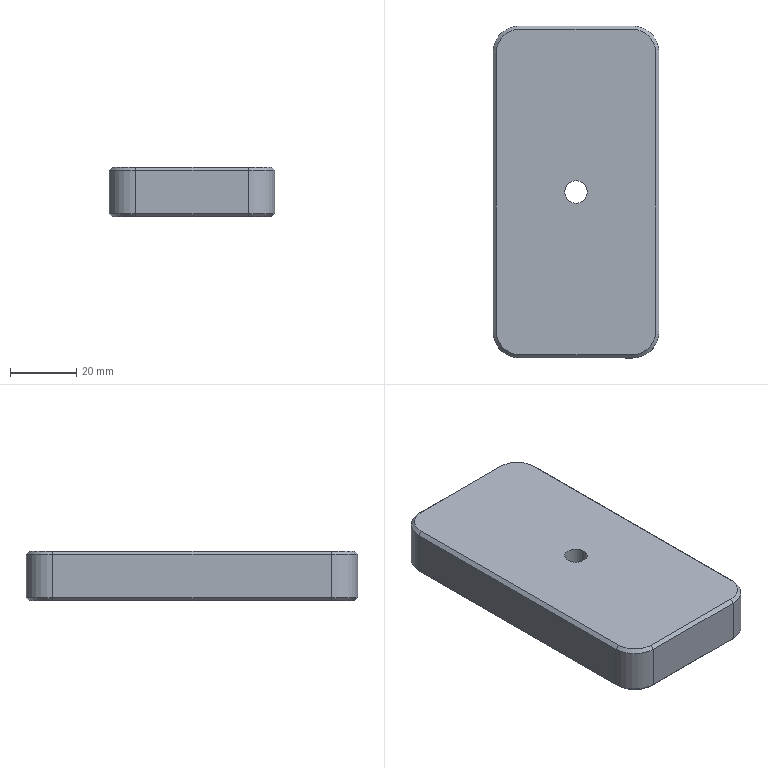Component | SolidWorks | 01-01FrameBody-1_02LowerRackSpacer-5 | 1 solid | 28 faces | box 50 x 100 x 15 mm | volume 73347 mm3 | plane 14 | cone 8 | cylinder 6 | commonest cylinder face diameters 16 x4 6.8 x2 | material 4040 Square Tube
build123d program:
from build123d import *

# Parameters (mm, degrees)
SKETCH1_W           = 50
SKETCH1_H           = 100
BOSS_EXTRUDE1_DEPTH = 15
M8_TAPPED_HOLE1_D   = 6.8
FILLET1_R           = 8
CHAMFER1_SIZE       = 1


with BuildPart() as part:
    # Sketch1 → Boss-Extrude1 (new body)
    with BuildSketch(Plane.XY):
        Rectangle(SKETCH1_W, SKETCH1_H)
    extrude(amount=BOSS_EXTRUDE1_DEPTH)

    # M8 Tapped Hole1 (through all)
    with Locations(Plane.XY.offset(15)):
        with Locations((0, 0)):
            Hole(M8_TAPPED_HOLE1_D / 2)

    # Fillet1
    fillet1_edges = [part.edges().sort_by_distance(p)[0] for p in [
        (25, -50, 7.5),
        (-25, -50, 7.5),
        (-25, 50, 7.5),
        (25, 50, 7.5),
    ]]
    fillet(fillet1_edges, radius=FILLET1_R)

    # Chamfer1
    chamfer1_edges = [part.edges().sort_by_distance(p)[0] for p in [
        (-25, 0, 0),
        (-25, 0, 15),
        (25, 0, 0),
        (0, -50, 0),
        (0, 50, 0),
        (22.657, -47.657, 0),
        (-22.657, -47.657, 0),
        (22.657, 47.657, 0),
        (-22.657, 47.657, 0),
        (0, 50, 15),
        (25, 0, 15),
        (0, -50, 15),
        (22.657, -47.657, 15),
        (-22.657, -47.657, 15),
        (22.657, 47.657, 15),
        (-22.657, 47.657, 15),
    ]]
    chamfer(chamfer1_edges, length=CHAMFER1_SIZE)


solid = part.part

# Placed as in the assembly
solid = solid.moved(Location((-25, 670, 625), (0, 0, 0)))
STEP:
#1=COLOUR_RGB('',0.7922,0.8196,0.9333);
#2=FILL_AREA_STYLE_COLOUR('',#1);
#3=FILL_AREA_STYLE('',(#2));
#4=SURFACE_STYLE_FILL_AREA(#3);
#5=SURFACE_SIDE_STYLE('',(#4));
#6=SURFACE_STYLE_USAGE(.BOTH.,#5);
#7=PRESENTATION_STYLE_ASSIGNMENT((#6));
#8=CARTESIAN_POINT('',(-1.118,26.378,25.197));
#9=VERTEX_POINT('',#8);
#10=CARTESIAN_POINT('',(-0.8504,26.378,25.197));
#11=VERTEX_POINT('',#10);
#12=CARTESIAN_POINT('',(-0.9843,26.378,25.197));
#13=DIRECTION('',(0.,-0.,-1.));
#14=DIRECTION('',(1.,0.,0.));
#15=AXIS2_PLACEMENT_3D('',#12,#13,#14);
#16=CIRCLE('',#15,0.1339);
#17=EDGE_CURVE('',#9,#11,#16,.T.);
#18=ORIENTED_EDGE('',*,*,#17,.F.);
#19=CARTESIAN_POINT('',(-1.118,26.378,24.606));
#20=VERTEX_POINT('',#19);
#21=CARTESIAN_POINT('',(-1.118,26.378,24.606));
#22=DIRECTION('',(0.,-0.,-1.));
#23=VECTOR('',#22,39.37);
#24=LINE('',#21,#23);
#25=EDGE_CURVE('',#9,#20,#24,.T.);
#26=ORIENTED_EDGE('',*,*,#25,.T.);
#27=CARTESIAN_POINT('',(-0.8504,26.378,24.606));
#28=VERTEX_POINT('',#27);
#29=CARTESIAN_POINT('',(-0.9843,26.378,24.606));
#30=DIRECTION('',(0.,-0.,-1.));
#31=DIRECTION('',(1.,0.,0.));
#32=AXIS2_PLACEMENT_3D('',#29,#30,#31);
#33=CIRCLE('',#32,0.1339);
#34=EDGE_CURVE('',#20,#28,#33,.T.);
#35=ORIENTED_EDGE('',*,*,#34,.T.);
#36=CARTESIAN_POINT('',(-0.8504,26.378,24.606));
#37=DIRECTION('',(0.,-0.,-1.));
#38=VECTOR('',#37,39.37);
#39=LINE('',#36,#38);
#40=EDGE_CURVE('',#11,#28,#39,.T.);
#41=ORIENTED_EDGE('',*,*,#40,.F.);
#42=EDGE_LOOP('',(#18,#26,#35,#41));
#43=FACE_OUTER_BOUND('',#42,.T.);
#44=CARTESIAN_POINT('',(-0.9843,26.378,24.606));
#45=DIRECTION('',(0.,-0.,-1.));
#46=DIRECTION('',(1.,0.,0.));
#47=AXIS2_PLACEMENT_3D('',#44,#45,#46);
#48=CYLINDRICAL_SURFACE('',#47,0.1339);
#49=ADVANCED_FACE('',(#43),#48,.F.);
#50=CARTESIAN_POINT('',(-0.,24.724,25.157));
#51=VERTEX_POINT('',#50);
#52=CARTESIAN_POINT('',(-0.,24.724,24.646));
#53=VERTEX_POINT('',#52);
#54=CARTESIAN_POINT('',(-0.,24.724,24.606));
#55=DIRECTION('',(0.,-0.,-1.));
#56=VECTOR('',#55,39.37);
#57=LINE('',#54,#56);
#58=EDGE_CURVE('',#51,#53,#57,.T.);
#59=ORIENTED_EDGE('',*,*,#58,.T.);
#60=CARTESIAN_POINT('',(-0.,28.031,24.646));
#61=VERTEX_POINT('',#60);
#62=CARTESIAN_POINT('',(-0.,28.031,24.646));
#63=DIRECTION('',(0.,1.,-0.));
#64=VECTOR('',#63,39.37);
#65=LINE('',#62,#64);
#66=EDGE_CURVE('',#53,#61,#65,.T.);
#67=ORIENTED_EDGE('',*,*,#66,.T.);
#68=CARTESIAN_POINT('',(-0.,28.031,25.157));
#69=VERTEX_POINT('',#68);
#70=CARTESIAN_POINT('',(-0.,28.031,24.606));
#71=DIRECTION('',(-0.,0.,1.));
#72=VECTOR('',#71,39.37);
#73=LINE('',#70,#72);
#74=EDGE_CURVE('',#61,#69,#73,.T.);
#75=ORIENTED_EDGE('',*,*,#74,.T.);
#76=CARTESIAN_POINT('',(-0.,24.409,25.157));
#77=DIRECTION('',(-0.,-1.,0.));
#78=VECTOR('',#77,39.37);
#79=LINE('',#76,#78);
#80=EDGE_CURVE('',#69,#51,#79,.T.);
#81=ORIENTED_EDGE('',*,*,#80,.T.);
#82=EDGE_LOOP('',(#59,#67,#75,#81));
#83=FACE_OUTER_BOUND('',#82,.T.);
#84=CARTESIAN_POINT('',(-0.,24.409,24.606));
#85=DIRECTION('',(-1.,0.,-0.));
#86=DIRECTION('',(0.,1.,-0.));
#87=AXIS2_PLACEMENT_3D('',#84,#85,#86);
#88=PLANE('',#87);
#89=ADVANCED_FACE('',(#83),#88,.F.);
#90=CARTESIAN_POINT('',(-1.654,24.409,25.157));
#91=VERTEX_POINT('',#90);
#92=CARTESIAN_POINT('',(-1.654,24.409,24.646));
#93=VERTEX_POINT('',#92);
#94=CARTESIAN_POINT('',(-1.654,24.409,24.606));
#95=DIRECTION('',(0.,-0.,-1.));
#96=VECTOR('',#95,39.37);
#97=LINE('',#94,#96);
#98=EDGE_CURVE('',#91,#93,#97,.T.);
#99=ORIENTED_EDGE('',*,*,#98,.T.);
#100=CARTESIAN_POINT('',(-0.315,24.409,24.646));
#101=VERTEX_POINT('',#100);
#102=CARTESIAN_POINT('',(-0.315,24.409,24.646));
#103=DIRECTION('',(1.,-0.,0.));
#104=VECTOR('',#103,39.37);
#105=LINE('',#102,#104);
#106=EDGE_CURVE('',#93,#101,#105,.T.);
#107=ORIENTED_EDGE('',*,*,#106,.T.);
#108=CARTESIAN_POINT('',(-0.315,24.409,25.157));
#109=VERTEX_POINT('',#108);
#110=CARTESIAN_POINT('',(-0.315,24.409,24.606));
#111=DIRECTION('',(-0.,0.,1.));
#112=VECTOR('',#111,39.37);
#113=LINE('',#110,#112);
#114=EDGE_CURVE('',#101,#109,#113,.T.);
#115=ORIENTED_EDGE('',*,*,#114,.T.);
#116=CARTESIAN_POINT('',(-1.969,24.409,25.157));
#117=DIRECTION('',(-1.,0.,-0.));
#118=VECTOR('',#117,39.37);
#119=LINE('',#116,#118);
#120=EDGE_CURVE('',#109,#91,#119,.T.);
#121=ORIENTED_EDGE('',*,*,#120,.T.);
#122=EDGE_LOOP('',(#99,#107,#115,#121));
#123=FACE_OUTER_BOUND('',#122,.T.);
#124=CARTESIAN_POINT('',(-1.969,24.409,24.606));
#125=DIRECTION('',(0.,1.,-0.));
#126=DIRECTION('',(-0.,0.,1.));
#127=AXIS2_PLACEMENT_3D('',#124,#125,#126);
#128=PLANE('',#127);
#129=ADVANCED_FACE('',(#123),#128,.F.);
#130=CARTESIAN_POINT('',(-1.969,28.031,25.157));
#131=VERTEX_POINT('',#130);
#132=CARTESIAN_POINT('',(-1.969,28.031,24.646));
#133=VERTEX_POINT('',#132);
#134=CARTESIAN_POINT('',(-1.969,28.031,24.606));
#135=DIRECTION('',(0.,-0.,-1.));
#136=VECTOR('',#135,39.37);
#137=LINE('',#134,#136);
#138=EDGE_CURVE('',#131,#133,#137,.T.);
#139=ORIENTED_EDGE('',*,*,#138,.T.);
#140=CARTESIAN_POINT('',(-1.969,24.724,24.646));
#141=VERTEX_POINT('',#140);
#142=CARTESIAN_POINT('',(-1.969,24.724,24.646));
#143=DIRECTION('',(-0.,-1.,0.));
#144=VECTOR('',#143,39.37);
#145=LINE('',#142,#144);
#146=EDGE_CURVE('',#133,#141,#145,.T.);
#147=ORIENTED_EDGE('',*,*,#146,.T.);
#148=CARTESIAN_POINT('',(-1.969,24.724,25.157));
#149=VERTEX_POINT('',#148);
#150=CARTESIAN_POINT('',(-1.969,24.724,24.606));
#151=DIRECTION('',(-0.,0.,1.));
#152=VECTOR('',#151,39.37);
#153=LINE('',#150,#152);
#154=EDGE_CURVE('',#141,#149,#153,.T.);
#155=ORIENTED_EDGE('',*,*,#154,.T.);
#156=CARTESIAN_POINT('',(-1.969,24.409,25.157));
#157=DIRECTION('',(0.,1.,-0.));
#158=VECTOR('',#157,39.37);
#159=LINE('',#156,#158);
#160=EDGE_CURVE('',#149,#131,#159,.T.);
#161=ORIENTED_EDGE('',*,*,#160,.T.);
#162=EDGE_LOOP('',(#139,#147,#155,#161));
#163=FACE_OUTER_BOUND('',#162,.T.);
#164=CARTESIAN_POINT('',(-1.969,24.409,24.606));
#165=DIRECTION('',(1.,-0.,0.));
#166=DIRECTION('',(-0.,-1.,0.));
#167=AXIS2_PLACEMENT_3D('',#164,#165,#166);
#168=PLANE('',#167);
#169=ADVANCED_FACE('',(#163),#168,.F.);
#170=CARTESIAN_POINT('',(-0.315,28.346,25.157));
#171=VERTEX_POINT('',#170);
#172=CARTESIAN_POINT('',(-0.315,28.346,24.646));
#173=VERTEX_POINT('',#172);
#174=CARTESIAN_POINT('',(-0.315,28.346,24.606));
#175=DIRECTION('',(0.,-0.,-1.));
#176=VECTOR('',#175,39.37);
#177=LINE('',#174,#176);
#178=EDGE_CURVE('',#171,#173,#177,.T.);
#179=ORIENTED_EDGE('',*,*,#178,.T.);
#180=CARTESIAN_POINT('',(-1.654,28.346,24.646));
#181=VERTEX_POINT('',#180);
#182=CARTESIAN_POINT('',(-1.654,28.346,24.646));
#183=DIRECTION('',(-1.,0.,-0.));
#184=VECTOR('',#183,39.37);
#185=LINE('',#182,#184);
#186=EDGE_CURVE('',#173,#181,#185,.T.);
#187=ORIENTED_EDGE('',*,*,#186,.T.);
#188=CARTESIAN_POINT('',(-1.654,28.346,25.157));
#189=VERTEX_POINT('',#188);
#190=CARTESIAN_POINT('',(-1.654,28.346,24.606));
#191=DIRECTION('',(-0.,0.,1.));
#192=VECTOR('',#191,39.37);
#193=LINE('',#190,#192);
#194=EDGE_CURVE('',#181,#189,#193,.T.);
#195=ORIENTED_EDGE('',*,*,#194,.T.);
#196=CARTESIAN_POINT('',(-1.969,28.346,25.157));
#197=DIRECTION('',(1.,-0.,0.));
#198=VECTOR('',#197,39.37);
#199=LINE('',#196,#198);
#200=EDGE_CURVE('',#189,#171,#199,.T.);
#201=ORIENTED_EDGE('',*,*,#200,.T.);
#202=EDGE_LOOP('',(#179,#187,#195,#201));
#203=FACE_OUTER_BOUND('',#202,.T.);
#204=CARTESIAN_POINT('',(-1.969,28.346,24.606));
#205=DIRECTION('',(-0.,-1.,0.));
#206=DIRECTION('',(0.,-0.,-1.));
#207=AXIS2_PLACEMENT_3D('',#204,#205,#206);
#208=PLANE('',#207);
#209=ADVANCED_FACE('',(#203),#208,.F.);
#210=CARTESIAN_POINT('',(-1.654,28.307,24.606));
#211=VERTEX_POINT('',#210);
#212=CARTESIAN_POINT('',(-0.315,28.307,24.606));
#213=VERTEX_POINT('',#212);
#214=CARTESIAN_POINT('',(-0.315,28.307,24.606));
#215=DIRECTION('',(1.,-0.,0.));
#216=VECTOR('',#215,39.37);
#217=LINE('',#214,#216);
#218=EDGE_CURVE('',#211,#213,#217,.T.);
#219=ORIENTED_EDGE('',*,*,#218,.T.);
#220=CARTESIAN_POINT('',(-0.03937,28.031,24.606));
#221=VERTEX_POINT('',#220);
#222=CARTESIAN_POINT('',(-0.315,28.031,24.606));
#223=DIRECTION('',(0.,-0.,-1.));
#224=DIRECTION('',(1.,0.,0.));
#225=AXIS2_PLACEMENT_3D('',#222,#223,#224);
#226=CIRCLE('',#225,0.2756);
#227=EDGE_CURVE('',#213,#221,#226,.T.);
#228=ORIENTED_EDGE('',*,*,#227,.T.);
#229=CARTESIAN_POINT('',(-0.03937,24.724,24.606));
#230=VERTEX_POINT('',#229);
#231=CARTESIAN_POINT('',(-0.03937,24.724,24.606));
#232=DIRECTION('',(-0.,-1.,0.));
#233=VECTOR('',#232,39.37);
#234=LINE('',#231,#233);
#235=EDGE_CURVE('',#221,#230,#234,.T.);
#236=ORIENTED_EDGE('',*,*,#235,.T.);
#237=CARTESIAN_POINT('',(-0.315,24.449,24.606));
#238=VERTEX_POINT('',#237);
#239=CARTESIAN_POINT('',(-0.315,24.724,24.606));
#240=DIRECTION('',(0.,-0.,-1.));
#241=DIRECTION('',(1.,0.,0.));
#242=AXIS2_PLACEMENT_3D('',#239,#240,#241);
#243=CIRCLE('',#242,0.2756);
#244=EDGE_CURVE('',#230,#238,#243,.T.);
#245=ORIENTED_EDGE('',*,*,#244,.T.);
#246=CARTESIAN_POINT('',(-1.654,24.449,24.606));
#247=VERTEX_POINT('',#246);
#248=CARTESIAN_POINT('',(-1.654,24.449,24.606));
#249=DIRECTION('',(-1.,0.,-0.));
#250=VECTOR('',#249,39.37);
#251=LINE('',#248,#250);
#252=EDGE_CURVE('',#238,#247,#251,.T.);
#253=ORIENTED_EDGE('',*,*,#252,.T.);
#254=CARTESIAN_POINT('',(-1.929,24.724,24.606));
#255=VERTEX_POINT('',#254);
#256=CARTESIAN_POINT('',(-1.654,24.724,24.606));
#257=DIRECTION('',(0.,-0.,-1.));
#258=DIRECTION('',(1.,0.,0.));
#259=AXIS2_PLACEMENT_3D('',#256,#257,#258);
#260=CIRCLE('',#259,0.2756);
#261=EDGE_CURVE('',#247,#255,#260,.T.);
#262=ORIENTED_EDGE('',*,*,#261,.T.);
#263=CARTESIAN_POINT('',(-1.929,28.031,24.606));
#264=VERTEX_POINT('',#263);
#265=CARTESIAN_POINT('',(-1.929,28.031,24.606));
#266=DIRECTION('',(0.,1.,-0.));
#267=VECTOR('',#266,39.37);
#268=LINE('',#265,#267);
#269=EDGE_CURVE('',#255,#264,#268,.T.);
#270=ORIENTED_EDGE('',*,*,#269,.T.);
#271=CARTESIAN_POINT('',(-1.654,28.031,24.606));
#272=DIRECTION('',(0.,-0.,-1.));
#273=DIRECTION('',(1.,0.,0.));
#274=AXIS2_PLACEMENT_3D('',#271,#272,#273);
#275=CIRCLE('',#274,0.2756);
#276=EDGE_CURVE('',#264,#211,#275,.T.);
#277=ORIENTED_EDGE('',*,*,#276,.T.);
#278=EDGE_LOOP('',(#219,#228,#236,#245,#253,#262,#270,#277));
#279=FACE_OUTER_BOUND('',#278,.T.);
#280=CARTESIAN_POINT('',(-0.9843,26.378,24.606));
#281=DIRECTION('',(0.,-0.,-1.));
#282=DIRECTION('',(1.,0.,0.));
#283=AXIS2_PLACEMENT_3D('',#280,#281,#282);
#284=CIRCLE('',#283,0.1339);
#285=EDGE_CURVE('',#28,#20,#284,.T.);
#286=ORIENTED_EDGE('',*,*,#285,.F.);
#287=ORIENTED_EDGE('',*,*,#34,.F.);
#288=EDGE_LOOP('',(#286,#287));
#289=FACE_BOUND('',#288,.T.);
#290=CARTESIAN_POINT('',(-0.,28.346,24.606));
#291=DIRECTION('',(0.,-0.,-1.));
#292=DIRECTION('',(1.,-0.,0.));
#293=AXIS2_PLACEMENT_3D('',#290,#291,#292);
#294=PLANE('',#293);
#295=ADVANCED_FACE('',(#279,#289),#294,.T.);
#296=CARTESIAN_POINT('',(-1.654,24.449,25.197));
#297=VERTEX_POINT('',#296);
#298=CARTESIAN_POINT('',(-0.315,24.449,25.197));
#299=VERTEX_POINT('',#298);
#300=CARTESIAN_POINT('',(-0.,24.449,25.197));
#301=DIRECTION('',(1.,-0.,0.));
#302=VECTOR('',#301,39.37);
#303=LINE('',#300,#302);
#304=EDGE_CURVE('',#297,#299,#303,.T.);
#305=ORIENTED_EDGE('',*,*,#304,.T.);
#306=CARTESIAN_POINT('',(-0.03937,24.724,25.197));
#307=VERTEX_POINT('',#306);
#308=CARTESIAN_POINT('',(-0.315,24.724,25.197));
#309=DIRECTION('',(-0.,0.,1.));
#310=DIRECTION('',(1.,0.,0.));
#311=AXIS2_PLACEMENT_3D('',#308,#309,#310);
#312=CIRCLE('',#311,0.2756);
#313=EDGE_CURVE('',#299,#307,#312,.T.);
#314=ORIENTED_EDGE('',*,*,#313,.T.);
#315=CARTESIAN_POINT('',(-0.03937,28.031,25.197));
#316=VERTEX_POINT('',#315);
#317=CARTESIAN_POINT('',(-0.03937,28.346,25.197));
#318=DIRECTION('',(0.,1.,-0.));
#319=VECTOR('',#318,39.37);
#320=LINE('',#317,#319);
#321=EDGE_CURVE('',#307,#316,#320,.T.);
#322=ORIENTED_EDGE('',*,*,#321,.T.);
#323=CARTESIAN_POINT('',(-0.315,28.307,25.197));
#324=VERTEX_POINT('',#323);
#325=CARTESIAN_POINT('',(-0.315,28.031,25.197));
#326=DIRECTION('',(-0.,0.,1.));
#327=DIRECTION('',(1.,0.,0.));
#328=AXIS2_PLACEMENT_3D('',#325,#326,#327);
#329=CIRCLE('',#328,0.2756);
#330=EDGE_CURVE('',#316,#324,#329,.T.);
#331=ORIENTED_EDGE('',*,*,#330,.T.);
#332=CARTESIAN_POINT('',(-1.654,28.307,25.197));
#333=VERTEX_POINT('',#332);
#334=CARTESIAN_POINT('',(-0.,28.307,25.197));
#335=DIRECTION('',(-1.,0.,-0.));
#336=VECTOR('',#335,39.37);
#337=LINE('',#334,#336);
#338=EDGE_CURVE('',#324,#333,#337,.T.);
#339=ORIENTED_EDGE('',*,*,#338,.T.);
#340=CARTESIAN_POINT('',(-1.929,28.031,25.197));
#341=VERTEX_POINT('',#340);
#342=CARTESIAN_POINT('',(-1.654,28.031,25.197));
#343=DIRECTION('',(-0.,0.,1.));
#344=DIRECTION('',(1.,0.,0.));
#345=AXIS2_PLACEMENT_3D('',#342,#343,#344);
#346=CIRCLE('',#345,0.2756);
#347=EDGE_CURVE('',#333,#341,#346,.T.);
#348=ORIENTED_EDGE('',*,*,#347,.T.);
#349=CARTESIAN_POINT('',(-1.929,24.724,25.197));
#350=VERTEX_POINT('',#349);
#351=CARTESIAN_POINT('',(-1.929,28.346,25.197));
#352=DIRECTION('',(-0.,-1.,0.));
#353=VECTOR('',#352,39.37);
#354=LINE('',#351,#353);
#355=EDGE_CURVE('',#341,#350,#354,.T.);
#356=ORIENTED_EDGE('',*,*,#355,.T.);
#357=CARTESIAN_POINT('',(-1.654,24.724,25.197));
#358=DIRECTION('',(-0.,0.,1.));
#359=DIRECTION('',(1.,0.,0.));
#360=AXIS2_PLACEMENT_3D('',#357,#358,#359);
#361=CIRCLE('',#360,0.2756);
#362=EDGE_CURVE('',#350,#297,#361,.T.);
#363=ORIENTED_EDGE('',*,*,#362,.T.);
#364=EDGE_LOOP('',(#305,#314,#322,#331,#339,#348,#356,#363));
#365=FACE_OUTER_BOUND('',#364,.T.);
#366=CARTESIAN_POINT('',(-0.9843,26.378,25.197));
#367=DIRECTION('',(0.,-0.,-1.));
#368=DIRECTION('',(1.,0.,0.));
#369=AXIS2_PLACEMENT_3D('',#366,#367,#368);
#370=CIRCLE('',#369,0.1339);
#371=EDGE_CURVE('',#11,#9,#370,.T.);
#372=ORIENTED_EDGE('',*,*,#371,.T.);
#373=ORIENTED_EDGE('',*,*,#17,.T.);
#374=EDGE_LOOP('',(#372,#373));
#375=FACE_BOUND('',#374,.T.);
#376=CARTESIAN_POINT('',(-0.,28.346,25.197));
#377=DIRECTION('',(0.,-0.,-1.));
#378=DIRECTION('',(1.,-0.,0.));
#379=AXIS2_PLACEMENT_3D('',#376,#377,#378);
#380=PLANE('',#379);
#381=ADVANCED_FACE('',(#365,#375),#380,.F.);
#382=ORIENTED_EDGE('',*,*,#25,.F.);
#383=ORIENTED_EDGE('',*,*,#371,.F.);
#384=ORIENTED_EDGE('',*,*,#40,.T.);
#385=ORIENTED_EDGE('',*,*,#285,.T.);
#386=EDGE_LOOP('',(#382,#383,#384,#385));
#387=FACE_OUTER_BOUND('',#386,.T.);
#388=CARTESIAN_POINT('',(-0.9843,26.378,24.606));
#389=DIRECTION('',(0.,-0.,-1.));
#390=DIRECTION('',(1.,0.,0.));
#391=AXIS2_PLACEMENT_3D('',#388,#389,#390);
#392=CYLINDRICAL_SURFACE('',#391,0.1339);
#393=ADVANCED_FACE('',(#387),#392,.F.);
#394=ORIENTED_EDGE('',*,*,#154,.F.);
#395=CARTESIAN_POINT('',(-1.654,24.724,24.646));
#396=DIRECTION('',(-0.,0.,1.));
#397=DIRECTION('',(1.,0.,0.));
#398=AXIS2_PLACEMENT_3D('',#395,#396,#397);
#399=CIRCLE('',#398,0.315);
#400=EDGE_CURVE('',#141,#93,#399,.T.);
#401=ORIENTED_EDGE('',*,*,#400,.T.);
#402=ORIENTED_EDGE('',*,*,#98,.F.);
#403=CARTESIAN_POINT('',(-1.654,24.724,25.157));
#404=DIRECTION('',(0.,-0.,-1.));
#405=DIRECTION('',(1.,0.,0.));
#406=AXIS2_PLACEMENT_3D('',#403,#404,#405);
#407=CIRCLE('',#406,0.315);
#408=EDGE_CURVE('',#91,#149,#407,.T.);
#409=ORIENTED_EDGE('',*,*,#408,.T.);
#410=EDGE_LOOP('',(#394,#401,#402,#409));
#411=FACE_OUTER_BOUND('',#410,.T.);
#412=CARTESIAN_POINT('',(-1.654,24.724,24.606));
#413=DIRECTION('',(-0.,0.,1.));
#414=DIRECTION('',(-1.,0.,0.));
#415=AXIS2_PLACEMENT_3D('',#412,#413,#414);
#416=CYLINDRICAL_SURFACE('',#415,0.315);
#417=ADVANCED_FACE('',(#411),#416,.T.);
#418=ORIENTED_EDGE('',*,*,#114,.F.);
#419=CARTESIAN_POINT('',(-0.315,24.724,24.646));
#420=DIRECTION('',(-0.,0.,1.));
#421=DIRECTION('',(1.,0.,0.));
#422=AXIS2_PLACEMENT_3D('',#419,#420,#421);
#423=CIRCLE('',#422,0.315);
#424=EDGE_CURVE('',#101,#53,#423,.T.);
#425=ORIENTED_EDGE('',*,*,#424,.T.);
#426=ORIENTED_EDGE('',*,*,#58,.F.);
#427=CARTESIAN_POINT('',(-0.315,24.724,25.157));
#428=DIRECTION('',(0.,-0.,-1.));
#429=DIRECTION('',(1.,0.,0.));
#430=AXIS2_PLACEMENT_3D('',#427,#428,#429);
#431=CIRCLE('',#430,0.315);
#432=EDGE_CURVE('',#51,#109,#431,.T.);
#433=ORIENTED_EDGE('',*,*,#432,.T.);
#434=EDGE_LOOP('',(#418,#425,#426,#433));
#435=FACE_OUTER_BOUND('',#434,.T.);
#436=CARTESIAN_POINT('',(-0.315,24.724,24.606));
#437=DIRECTION('',(-0.,0.,1.));
#438=DIRECTION('',(-1.,0.,0.));
#439=AXIS2_PLACEMENT_3D('',#436,#437,#438);
#440=CYLINDRICAL_SURFACE('',#439,0.315);
#441=ADVANCED_FACE('',(#435),#440,.T.);
#442=ORIENTED_EDGE('',*,*,#194,.F.);
#443=CARTESIAN_POINT('',(-1.654,28.031,24.646));
#444=DIRECTION('',(-0.,0.,1.));
#445=DIRECTION('',(1.,0.,0.));
#446=AXIS2_PLACEMENT_3D('',#443,#444,#445);
#447=CIRCLE('',#446,0.315);
#448=EDGE_CURVE('',#181,#133,#447,.T.);
#449=ORIENTED_EDGE('',*,*,#448,.T.);
#450=ORIENTED_EDGE('',*,*,#138,.F.);
#451=CARTESIAN_POINT('',(-1.654,28.031,25.157));
#452=DIRECTION('',(0.,-0.,-1.));
#453=DIRECTION('',(1.,0.,0.));
#454=AXIS2_PLACEMENT_3D('',#451,#452,#453);
#455=CIRCLE('',#454,0.315);
#456=EDGE_CURVE('',#131,#189,#455,.T.);
#457=ORIENTED_EDGE('',*,*,#456,.T.);
#458=EDGE_LOOP('',(#442,#449,#450,#457));
#459=FACE_OUTER_BOUND('',#458,.T.);
#460=CARTESIAN_POINT('',(-1.654,28.031,24.606));
#461=DIRECTION('',(-0.,0.,1.));
#462=DIRECTION('',(-1.,0.,0.));
#463=AXIS2_PLACEMENT_3D('',#460,#461,#462);
#464=CYLINDRICAL_SURFACE('',#463,0.315);
#465=ADVANCED_FACE('',(#459),#464,.T.);
#466=ORIENTED_EDGE('',*,*,#74,.F.);
#467=CARTESIAN_POINT('',(-0.315,28.031,24.646));
#468=DIRECTION('',(-0.,0.,1.));
#469=DIRECTION('',(1.,0.,0.));
#470=AXIS2_PLACEMENT_3D('',#467,#468,#469);
#471=CIRCLE('',#470,0.315);
#472=EDGE_CURVE('',#61,#173,#471,.T.);
#473=ORIENTED_EDGE('',*,*,#472,.T.);
#474=ORIENTED_EDGE('',*,*,#178,.F.);
#475=CARTESIAN_POINT('',(-0.315,28.031,25.157));
#476=DIRECTION('',(0.,-0.,-1.));
#477=DIRECTION('',(1.,0.,0.));
#478=AXIS2_PLACEMENT_3D('',#475,#476,#477);
#479=CIRCLE('',#478,0.315);
#480=EDGE_CURVE('',#171,#69,#479,.T.);
#481=ORIENTED_EDGE('',*,*,#480,.T.);
#482=EDGE_LOOP('',(#466,#473,#474,#481));
#483=FACE_OUTER_BOUND('',#482,.T.);
#484=CARTESIAN_POINT('',(-0.315,28.031,24.606));
#485=DIRECTION('',(-0.,0.,1.));
#486=DIRECTION('',(-1.,0.,0.));
#487=AXIS2_PLACEMENT_3D('',#484,#485,#486);
#488=CYLINDRICAL_SURFACE('',#487,0.315);
#489=ADVANCED_FACE('',(#483),#488,.T.);
#490=CARTESIAN_POINT('',(-1.654,24.409,24.646));
#491=DIRECTION('',(0.,0.7071,-0.7071));
#492=VECTOR('',#491,39.37);
#493=LINE('',#490,#492);
#494=EDGE_CURVE('',#93,#247,#493,.T.);
#495=ORIENTED_EDGE('',*,*,#494,.F.);
#496=ORIENTED_EDGE('',*,*,#400,.F.);
#497=CARTESIAN_POINT('',(-1.929,24.724,24.606));
#498=DIRECTION('',(-0.7071,0.,0.7071));
#499=VECTOR('',#498,39.37);
#500=LINE('',#497,#499);
#501=EDGE_CURVE('',#255,#141,#500,.T.);
#502=ORIENTED_EDGE('',*,*,#501,.F.);
#503=ORIENTED_EDGE('',*,*,#261,.F.);
#504=EDGE_LOOP('',(#495,#496,#502,#503));
#505=FACE_OUTER_BOUND('',#504,.T.);
#506=CARTESIAN_POINT('',(-1.654,24.724,24.606));
#507=DIRECTION('',(-0.,0.,1.));
#508=DIRECTION('',(-1.,0.,0.));
#509=AXIS2_PLACEMENT_3D('',#506,#507,#508);
#510=CONICAL_SURFACE('',#509,0.2756,0.7854);
#511=ADVANCED_FACE('',(#505),#510,.T.);
#512=ORIENTED_EDGE('',*,*,#501,.T.);
#513=ORIENTED_EDGE('',*,*,#146,.F.);
#514=CARTESIAN_POINT('',(-1.929,28.031,24.606));
#515=DIRECTION('',(-0.7071,0.,0.7071));
#516=VECTOR('',#515,39.37);
#517=LINE('',#514,#516);
#518=EDGE_CURVE('',#264,#133,#517,.T.);
#519=ORIENTED_EDGE('',*,*,#518,.F.);
#520=ORIENTED_EDGE('',*,*,#269,.F.);
#521=EDGE_LOOP('',(#512,#513,#519,#520));
#522=FACE_OUTER_BOUND('',#521,.T.);
#523=CARTESIAN_POINT('',(-1.929,28.346,24.606));
#524=DIRECTION('',(-0.7071,0.,-0.7071));
#525=DIRECTION('',(0.7071,-0.,-0.7071));
#526=AXIS2_PLACEMENT_3D('',#523,#524,#525);
#527=PLANE('',#526);
#528=ADVANCED_FACE('',(#522),#527,.T.);
#529=ORIENTED_EDGE('',*,*,#494,.T.);
#530=ORIENTED_EDGE('',*,*,#252,.F.);
#531=CARTESIAN_POINT('',(-0.315,24.409,24.646));
#532=DIRECTION('',(0.,0.7071,-0.7071));
#533=VECTOR('',#532,39.37);
#534=LINE('',#531,#533);
#535=EDGE_CURVE('',#101,#238,#534,.T.);
#536=ORIENTED_EDGE('',*,*,#535,.F.);
#537=ORIENTED_EDGE('',*,*,#106,.F.);
#538=EDGE_LOOP('',(#529,#530,#536,#537));
#539=FACE_OUTER_BOUND('',#538,.T.);
#540=CARTESIAN_POINT('',(-0.,24.449,24.606));
#541=DIRECTION('',(-0.,-0.7071,-0.7071));
#542=DIRECTION('',(0.,0.7071,-0.7071));
#543=AXIS2_PLACEMENT_3D('',#540,#541,#542);
#544=PLANE('',#543);
#545=ADVANCED_FACE('',(#539),#544,.T.);
#546=ORIENTED_EDGE('',*,*,#518,.T.);
#547=ORIENTED_EDGE('',*,*,#448,.F.);
#548=CARTESIAN_POINT('',(-1.654,28.307,24.606));
#549=DIRECTION('',(0.,0.7071,0.7071));
#550=VECTOR('',#549,39.37);
#551=LINE('',#548,#550);
#552=EDGE_CURVE('',#211,#181,#551,.T.);
#553=ORIENTED_EDGE('',*,*,#552,.F.);
#554=ORIENTED_EDGE('',*,*,#276,.F.);
#555=EDGE_LOOP('',(#546,#547,#553,#554));
#556=FACE_OUTER_BOUND('',#555,.T.);
#557=CARTESIAN_POINT('',(-1.654,28.031,24.606));
#558=DIRECTION('',(-0.,0.,1.));
#559=DIRECTION('',(-1.,0.,0.));
#560=AXIS2_PLACEMENT_3D('',#557,#558,#559);
#561=CONICAL_SURFACE('',#560,0.2756,0.7854);
#562=ADVANCED_FACE('',(#556),#561,.T.);
#563=ORIENTED_EDGE('',*,*,#535,.T.);
#564=ORIENTED_EDGE('',*,*,#244,.F.);
#565=CARTESIAN_POINT('',(-0.,24.724,24.646));
#566=DIRECTION('',(-0.7071,0.,-0.7071));
#567=VECTOR('',#566,39.37);
#568=LINE('',#565,#567);
#569=EDGE_CURVE('',#53,#230,#568,.T.);
#570=ORIENTED_EDGE('',*,*,#569,.F.);
#571=ORIENTED_EDGE('',*,*,#424,.F.);
#572=EDGE_LOOP('',(#563,#564,#570,#571));
#573=FACE_OUTER_BOUND('',#572,.T.);
#574=CARTESIAN_POINT('',(-0.315,24.724,24.606));
#575=DIRECTION('',(-0.,0.,1.));
#576=DIRECTION('',(-1.,0.,0.));
#577=AXIS2_PLACEMENT_3D('',#574,#575,#576);
#578=CONICAL_SURFACE('',#577,0.2756,0.7854);
#579=ADVANCED_FACE('',(#573),#578,.T.);
#580=ORIENTED_EDGE('',*,*,#552,.T.);
#581=ORIENTED_EDGE('',*,*,#186,.F.);
#582=CARTESIAN_POINT('',(-0.315,28.307,24.606));
#583=DIRECTION('',(0.,0.7071,0.7071));
#584=VECTOR('',#583,39.37);
#585=LINE('',#582,#584);
#586=EDGE_CURVE('',#213,#173,#585,.T.);
#587=ORIENTED_EDGE('',*,*,#586,.F.);
#588=ORIENTED_EDGE('',*,*,#218,.F.);
#589=EDGE_LOOP('',(#580,#581,#587,#588));
#590=FACE_OUTER_BOUND('',#589,.T.);
#591=CARTESIAN_POINT('',(-0.,28.307,24.606));
#592=DIRECTION('',(0.,0.7071,-0.7071));
#593=DIRECTION('',(0.,0.7071,0.7071));
#594=AXIS2_PLACEMENT_3D('',#591,#592,#593);
#595=PLANE('',#594);
#596=ADVANCED_FACE('',(#590),#595,.T.);
#597=ORIENTED_EDGE('',*,*,#569,.T.);
#598=ORIENTED_EDGE('',*,*,#235,.F.);
#599=CARTESIAN_POINT('',(-0.,28.031,24.646));
#600=DIRECTION('',(-0.7071,0.,-0.7071));
#601=VECTOR('',#600,39.37);
#602=LINE('',#599,#601);
#603=EDGE_CURVE('',#61,#221,#602,.T.);
#604=ORIENTED_EDGE('',*,*,#603,.F.);
#605=ORIENTED_EDGE('',*,*,#66,.F.);
#606=EDGE_LOOP('',(#597,#598,#604,#605));
#607=FACE_OUTER_BOUND('',#606,.T.);
#608=CARTESIAN_POINT('',(-0.03937,28.346,24.606));
#609=DIRECTION('',(0.7071,-0.,-0.7071));
#610=DIRECTION('',(0.7071,-0.,0.7071));
#611=AXIS2_PLACEMENT_3D('',#608,#609,#610);
#612=PLANE('',#611);
#613=ADVANCED_FACE('',(#607),#612,.T.);
#614=ORIENTED_EDGE('',*,*,#586,.T.);
#615=ORIENTED_EDGE('',*,*,#472,.F.);
#616=ORIENTED_EDGE('',*,*,#603,.T.);
#617=ORIENTED_EDGE('',*,*,#227,.F.);
#618=EDGE_LOOP('',(#614,#615,#616,#617));
#619=FACE_OUTER_BOUND('',#618,.T.);
#620=CARTESIAN_POINT('',(-0.315,28.031,24.606));
#621=DIRECTION('',(-0.,0.,1.));
#622=DIRECTION('',(-1.,0.,0.));
#623=AXIS2_PLACEMENT_3D('',#620,#621,#622);
#624=CONICAL_SURFACE('',#623,0.2756,0.7854);
#625=ADVANCED_FACE('',(#619),#624,.T.);
#626=CARTESIAN_POINT('',(-1.654,28.346,25.157));
#627=DIRECTION('',(-0.,-0.7071,0.7071));
#628=VECTOR('',#627,39.37);
#629=LINE('',#626,#628);
#630=EDGE_CURVE('',#189,#333,#629,.T.);
#631=ORIENTED_EDGE('',*,*,#630,.F.);
#632=ORIENTED_EDGE('',*,*,#456,.F.);
#633=CARTESIAN_POINT('',(-1.929,28.031,25.197));
#634=DIRECTION('',(-0.7071,0.,-0.7071));
#635=VECTOR('',#634,39.37);
#636=LINE('',#633,#635);
#637=EDGE_CURVE('',#341,#131,#636,.T.);
#638=ORIENTED_EDGE('',*,*,#637,.F.);
#639=ORIENTED_EDGE('',*,*,#347,.F.);
#640=EDGE_LOOP('',(#631,#632,#638,#639));
#641=FACE_OUTER_BOUND('',#640,.T.);
#642=CARTESIAN_POINT('',(-1.654,28.031,25.197));
#643=DIRECTION('',(0.,-0.,-1.));
#644=DIRECTION('',(1.,0.,0.));
#645=AXIS2_PLACEMENT_3D('',#642,#643,#644);
#646=CONICAL_SURFACE('',#645,0.2756,0.7854);
#647=ADVANCED_FACE('',(#641),#646,.T.);
#648=ORIENTED_EDGE('',*,*,#637,.T.);
#649=ORIENTED_EDGE('',*,*,#160,.F.);
#650=CARTESIAN_POINT('',(-1.929,24.724,25.197));
#651=DIRECTION('',(-0.7071,0.,-0.7071));
#652=VECTOR('',#651,39.37);
#653=LINE('',#650,#652);
#654=EDGE_CURVE('',#350,#149,#653,.T.);
#655=ORIENTED_EDGE('',*,*,#654,.F.);
#656=ORIENTED_EDGE('',*,*,#355,.F.);
#657=EDGE_LOOP('',(#648,#649,#655,#656));
#658=FACE_OUTER_BOUND('',#657,.T.);
#659=CARTESIAN_POINT('',(-1.969,24.409,25.157));
#660=DIRECTION('',(0.7071,-0.,-0.7071));
#661=DIRECTION('',(0.7071,-0.,0.7071));
#662=AXIS2_PLACEMENT_3D('',#659,#660,#661);
#663=PLANE('',#662);
#664=ADVANCED_FACE('',(#658),#663,.F.);
#665=ORIENTED_EDGE('',*,*,#630,.T.);
#666=ORIENTED_EDGE('',*,*,#338,.F.);
#667=CARTESIAN_POINT('',(-0.315,28.346,25.157));
#668=DIRECTION('',(-0.,-0.7071,0.7071));
#669=VECTOR('',#668,39.37);
#670=LINE('',#667,#669);
#671=EDGE_CURVE('',#171,#324,#670,.T.);
#672=ORIENTED_EDGE('',*,*,#671,.F.);
#673=ORIENTED_EDGE('',*,*,#200,.F.);
#674=EDGE_LOOP('',(#665,#666,#672,#673));
#675=FACE_OUTER_BOUND('',#674,.T.);
#676=CARTESIAN_POINT('',(-1.969,28.346,25.157));
#677=DIRECTION('',(-0.,-0.7071,-0.7071));
#678=DIRECTION('',(0.,0.7071,-0.7071));
#679=AXIS2_PLACEMENT_3D('',#676,#677,#678);
#680=PLANE('',#679);
#681=ADVANCED_FACE('',(#675),#680,.F.);
#682=ORIENTED_EDGE('',*,*,#654,.T.);
#683=ORIENTED_EDGE('',*,*,#408,.F.);
#684=CARTESIAN_POINT('',(-1.654,24.449,25.197));
#685=DIRECTION('',(-0.,-0.7071,-0.7071));
#686=VECTOR('',#685,39.37);
#687=LINE('',#684,#686);
#688=EDGE_CURVE('',#297,#91,#687,.T.);
#689=ORIENTED_EDGE('',*,*,#688,.F.);
#690=ORIENTED_EDGE('',*,*,#362,.F.);
#691=EDGE_LOOP('',(#682,#683,#689,#690));
#692=FACE_OUTER_BOUND('',#691,.T.);
#693=CARTESIAN_POINT('',(-1.654,24.724,25.197));
#694=DIRECTION('',(0.,-0.,-1.));
#695=DIRECTION('',(1.,0.,0.));
#696=AXIS2_PLACEMENT_3D('',#693,#694,#695);
#697=CONICAL_SURFACE('',#696,0.2756,0.7854);
#698=ADVANCED_FACE('',(#692),#697,.T.);
#699=ORIENTED_EDGE('',*,*,#671,.T.);
#700=ORIENTED_EDGE('',*,*,#330,.F.);
#701=CARTESIAN_POINT('',(-0.,28.031,25.157));
#702=DIRECTION('',(-0.7071,0.,0.7071));
#703=VECTOR('',#702,39.37);
#704=LINE('',#701,#703);
#705=EDGE_CURVE('',#69,#316,#704,.T.);
#706=ORIENTED_EDGE('',*,*,#705,.F.);
#707=ORIENTED_EDGE('',*,*,#480,.F.);
#708=EDGE_LOOP('',(#699,#700,#706,#707));
#709=FACE_OUTER_BOUND('',#708,.T.);
#710=CARTESIAN_POINT('',(-0.315,28.031,25.197));
#711=DIRECTION('',(0.,-0.,-1.));
#712=DIRECTION('',(1.,0.,0.));
#713=AXIS2_PLACEMENT_3D('',#710,#711,#712);
#714=CONICAL_SURFACE('',#713,0.2756,0.7854);
#715=ADVANCED_FACE('',(#709),#714,.T.);
#716=ORIENTED_EDGE('',*,*,#688,.T.);
#717=ORIENTED_EDGE('',*,*,#120,.F.);
#718=CARTESIAN_POINT('',(-0.315,24.449,25.197));
#719=DIRECTION('',(-0.,-0.7071,-0.7071));
#720=VECTOR('',#719,39.37);
#721=LINE('',#718,#720);
#722=EDGE_CURVE('',#299,#109,#721,.T.);
#723=ORIENTED_EDGE('',*,*,#722,.F.);
#724=ORIENTED_EDGE('',*,*,#304,.F.);
#725=EDGE_LOOP('',(#716,#717,#723,#724));
#726=FACE_OUTER_BOUND('',#725,.T.);
#727=CARTESIAN_POINT('',(-1.969,24.409,25.157));
#728=DIRECTION('',(0.,0.7071,-0.7071));
#729=DIRECTION('',(0.,0.7071,0.7071));
#730=AXIS2_PLACEMENT_3D('',#727,#728,#729);
#731=PLANE('',#730);
#732=ADVANCED_FACE('',(#726),#731,.F.);
#733=ORIENTED_EDGE('',*,*,#705,.T.);
#734=ORIENTED_EDGE('',*,*,#321,.F.);
#735=CARTESIAN_POINT('',(-0.,24.724,25.157));
#736=DIRECTION('',(-0.7071,0.,0.7071));
#737=VECTOR('',#736,39.37);
#738=LINE('',#735,#737);
#739=EDGE_CURVE('',#51,#307,#738,.T.);
#740=ORIENTED_EDGE('',*,*,#739,.F.);
#741=ORIENTED_EDGE('',*,*,#80,.F.);
#742=EDGE_LOOP('',(#733,#734,#740,#741));
#743=FACE_OUTER_BOUND('',#742,.T.);
#744=CARTESIAN_POINT('',(-0.,24.409,25.157));
#745=DIRECTION('',(-0.7071,0.,-0.7071));
#746=DIRECTION('',(0.7071,-0.,-0.7071));
#747=AXIS2_PLACEMENT_3D('',#744,#745,#746);
#748=PLANE('',#747);
#749=ADVANCED_FACE('',(#743),#748,.F.);
#750=ORIENTED_EDGE('',*,*,#722,.T.);
#751=ORIENTED_EDGE('',*,*,#432,.F.);
#752=ORIENTED_EDGE('',*,*,#739,.T.);
#753=ORIENTED_EDGE('',*,*,#313,.F.);
#754=EDGE_LOOP('',(#750,#751,#752,#753));
#755=FACE_OUTER_BOUND('',#754,.T.);
#756=CARTESIAN_POINT('',(-0.315,24.724,25.197));
#757=DIRECTION('',(0.,-0.,-1.));
#758=DIRECTION('',(1.,0.,0.));
#759=AXIS2_PLACEMENT_3D('',#756,#757,#758);
#760=CONICAL_SURFACE('',#759,0.2756,0.7854);
#761=ADVANCED_FACE('',(#755),#760,.T.);
#762=CLOSED_SHELL('',(#49,#89,#129,#169,#209,#295,#381,#393,#417,#441,#465,#489,#511,#528,#545,#562,#579,#596,#613,#625,#647,#664,#681,#698,#715,#732,#749,#761));
#763=MANIFOLD_SOLID_BREP('',#762);
#764=STYLED_ITEM('',(#7),#763);
#765=(LENGTH_UNIT()NAMED_UNIT(*)SI_UNIT($,.METRE.));
#766=LENGTH_MEASURE_WITH_UNIT(LENGTH_MEASURE(0.0254),#765);
#767=DIMENSIONAL_EXPONENTS(1.,0.,0.,0.,0.,0.,0.);
#768=(CONVERSION_BASED_UNIT('',#766)LENGTH_UNIT()NAMED_UNIT(#767));
#769=UNCERTAINTY_MEASURE_WITH_UNIT(LENGTH_MEASURE(0.00001),#768,'','');
#770=(NAMED_UNIT(*)PLANE_ANGLE_UNIT()SI_UNIT($,.RADIAN.));
#771=(NAMED_UNIT(*)SI_UNIT($,.STERADIAN.)SOLID_ANGLE_UNIT());
#772=(GEOMETRIC_REPRESENTATION_CONTEXT(3)GLOBAL_UNCERTAINTY_ASSIGNED_CONTEXT((#769))GLOBAL_UNIT_ASSIGNED_CONTEXT((#768,#770,#771))REPRESENTATION_CONTEXT('',''));
#773=MECHANICAL_DESIGN_GEOMETRIC_PRESENTATION_REPRESENTATION('',(#764),#772);
#774=CARTESIAN_POINT('',(0.,0.,0.));
#775=DIRECTION('',(0.,0.,1.));
#776=DIRECTION('',(1.,0.,0.));
#777=AXIS2_PLACEMENT_3D('',#774,#775,#776);
#778=(LENGTH_UNIT()NAMED_UNIT(*)SI_UNIT($,.METRE.));
#779=LENGTH_MEASURE_WITH_UNIT(LENGTH_MEASURE(0.0254),#778);
#780=DIMENSIONAL_EXPONENTS(1.,0.,0.,0.,0.,0.,0.);
#781=(CONVERSION_BASED_UNIT('',#779)LENGTH_UNIT()NAMED_UNIT(#780));
#782=UNCERTAINTY_MEASURE_WITH_UNIT(LENGTH_MEASURE(0.00001),#781,'','');
#783=(NAMED_UNIT(*)PLANE_ANGLE_UNIT()SI_UNIT($,.RADIAN.));
#784=(NAMED_UNIT(*)SI_UNIT($,.STERADIAN.)SOLID_ANGLE_UNIT());
#785=(GEOMETRIC_REPRESENTATION_CONTEXT(3)GLOBAL_UNCERTAINTY_ASSIGNED_CONTEXT((#782))GLOBAL_UNIT_ASSIGNED_CONTEXT((#781,#783,#784))REPRESENTATION_CONTEXT('',''));
#786=ADVANCED_BREP_SHAPE_REPRESENTATION('',(#763,#777),#785);
#787=PRESENTATION_LAYER_ASSIGNMENT('','',(#764));